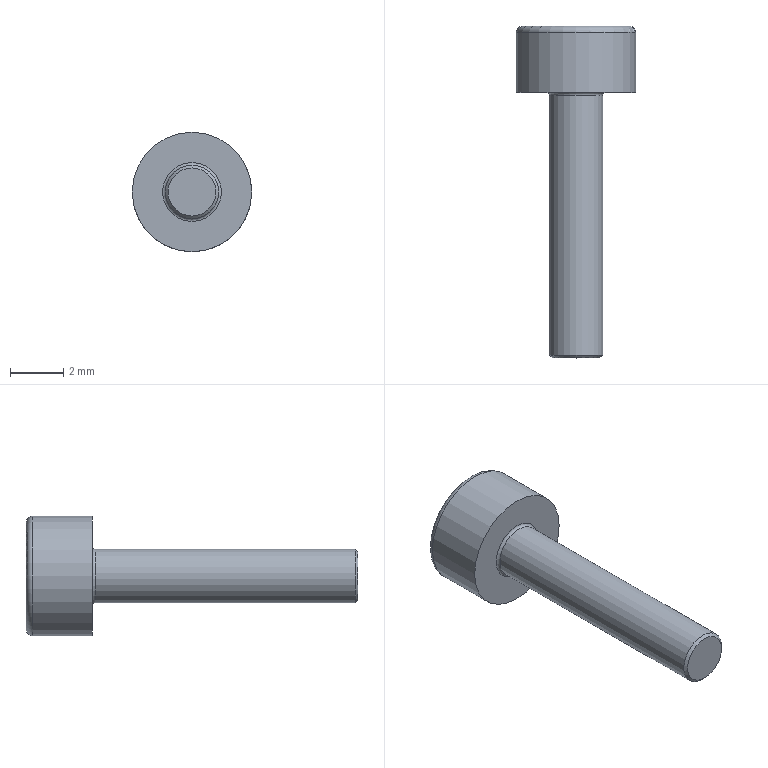Component | NX | SCREW_M2_5X10 | 1 solid | 27 faces | volume 65 mm3 | plane 15 | cone 8 | cylinder 2 | torus 2 | commonest cylinder face diameters 2.013 x1 4.5 x1